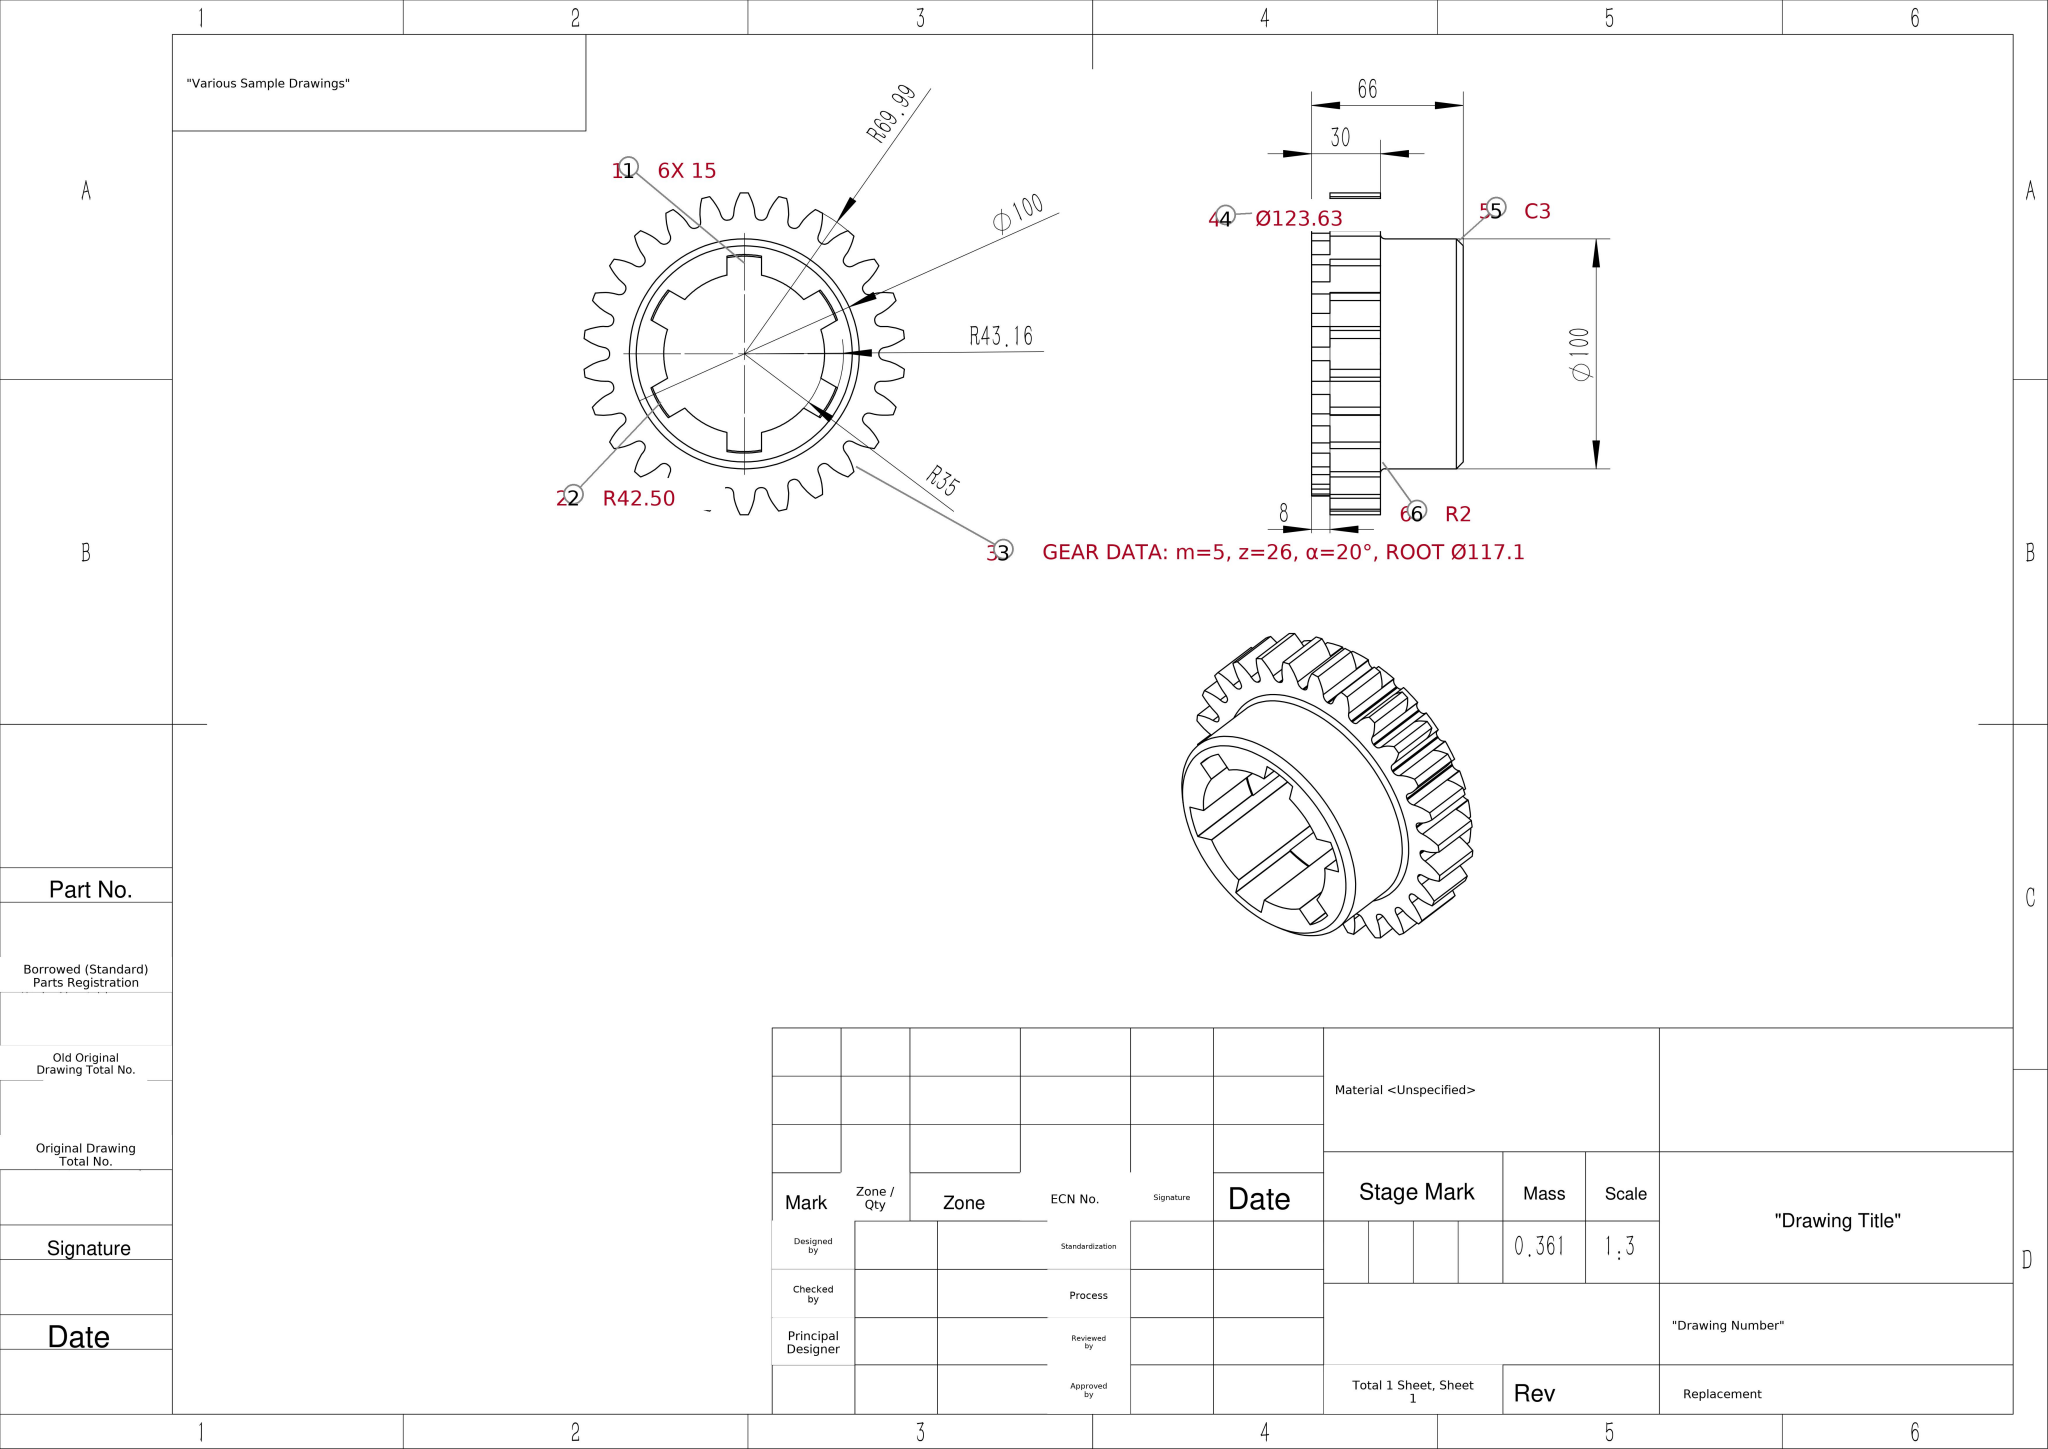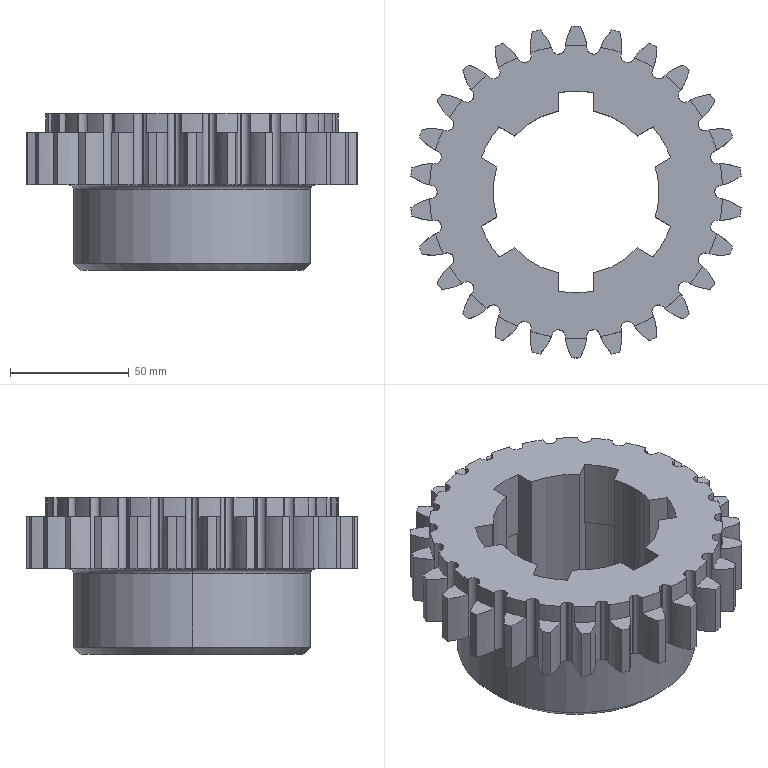Part | SolidWorks | mm | 1 solid | 308 faces | box 139.34 x 139.98 x 66 mm | volume 361067 mm3 | spline 104 | cylinder 101 | plane 99 | cone 2 | torus 2 | commonest cylinder face diameters 0.2 x28 139.98 x26 123.627 x26 70 x7 85 x6 86.313 x6 100 x2